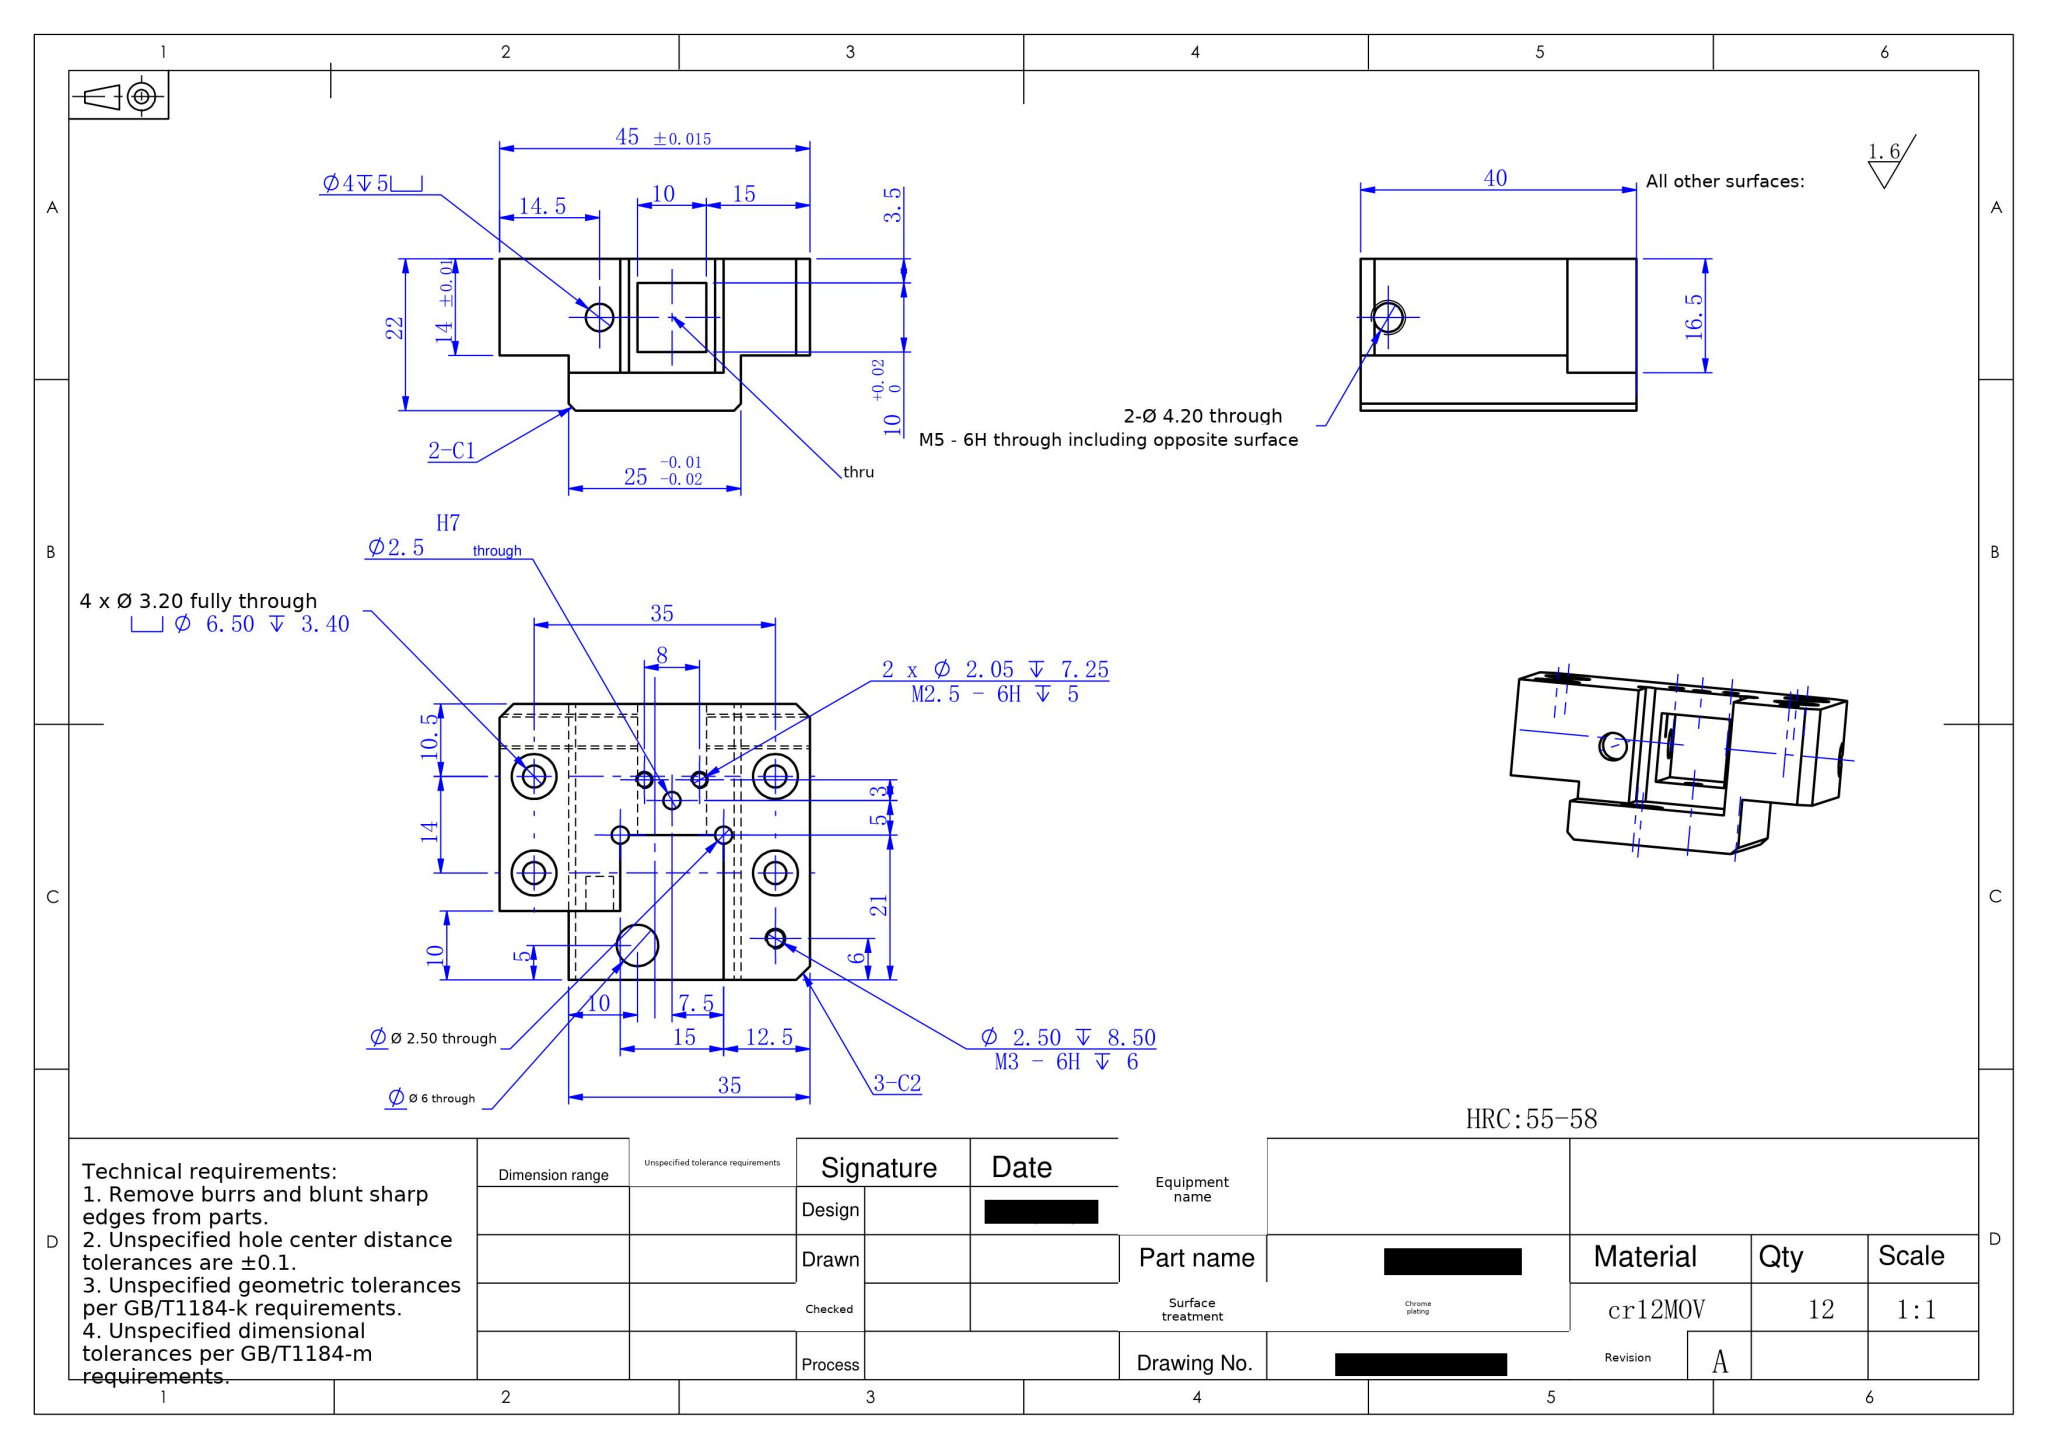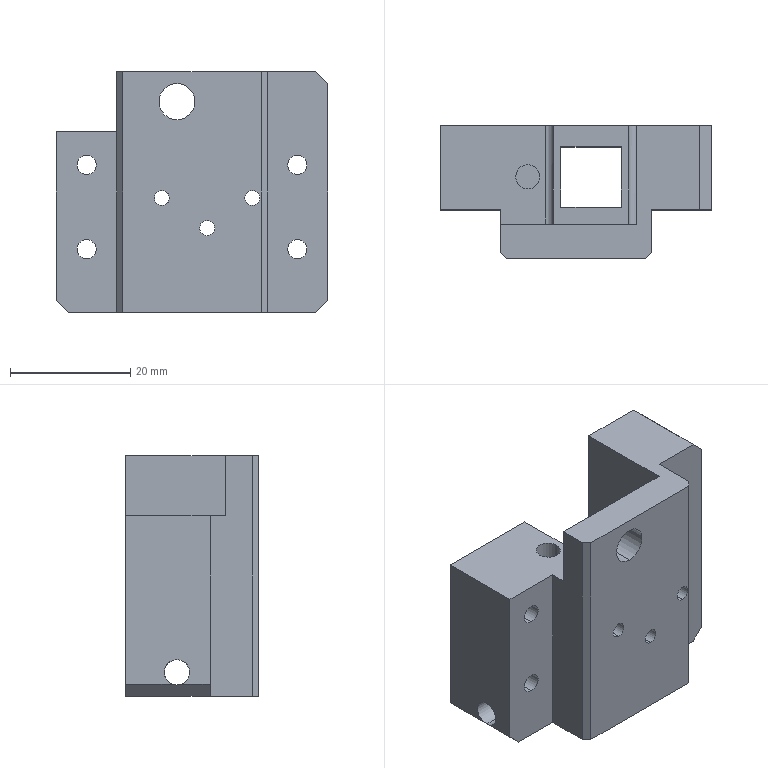Part | SolidWorks | mm | material cr12MOV | 1 solid | 71 faces | box 45 x 22 x 40 mm | volume 21545 mm3 | cylinder 38 | plane 29 | cone 4 | commonest cylinder face diameters 2.5 x10 6.5 x8 3.2 x8 2.05 x4 4.2 x4 6 x2 4 x2